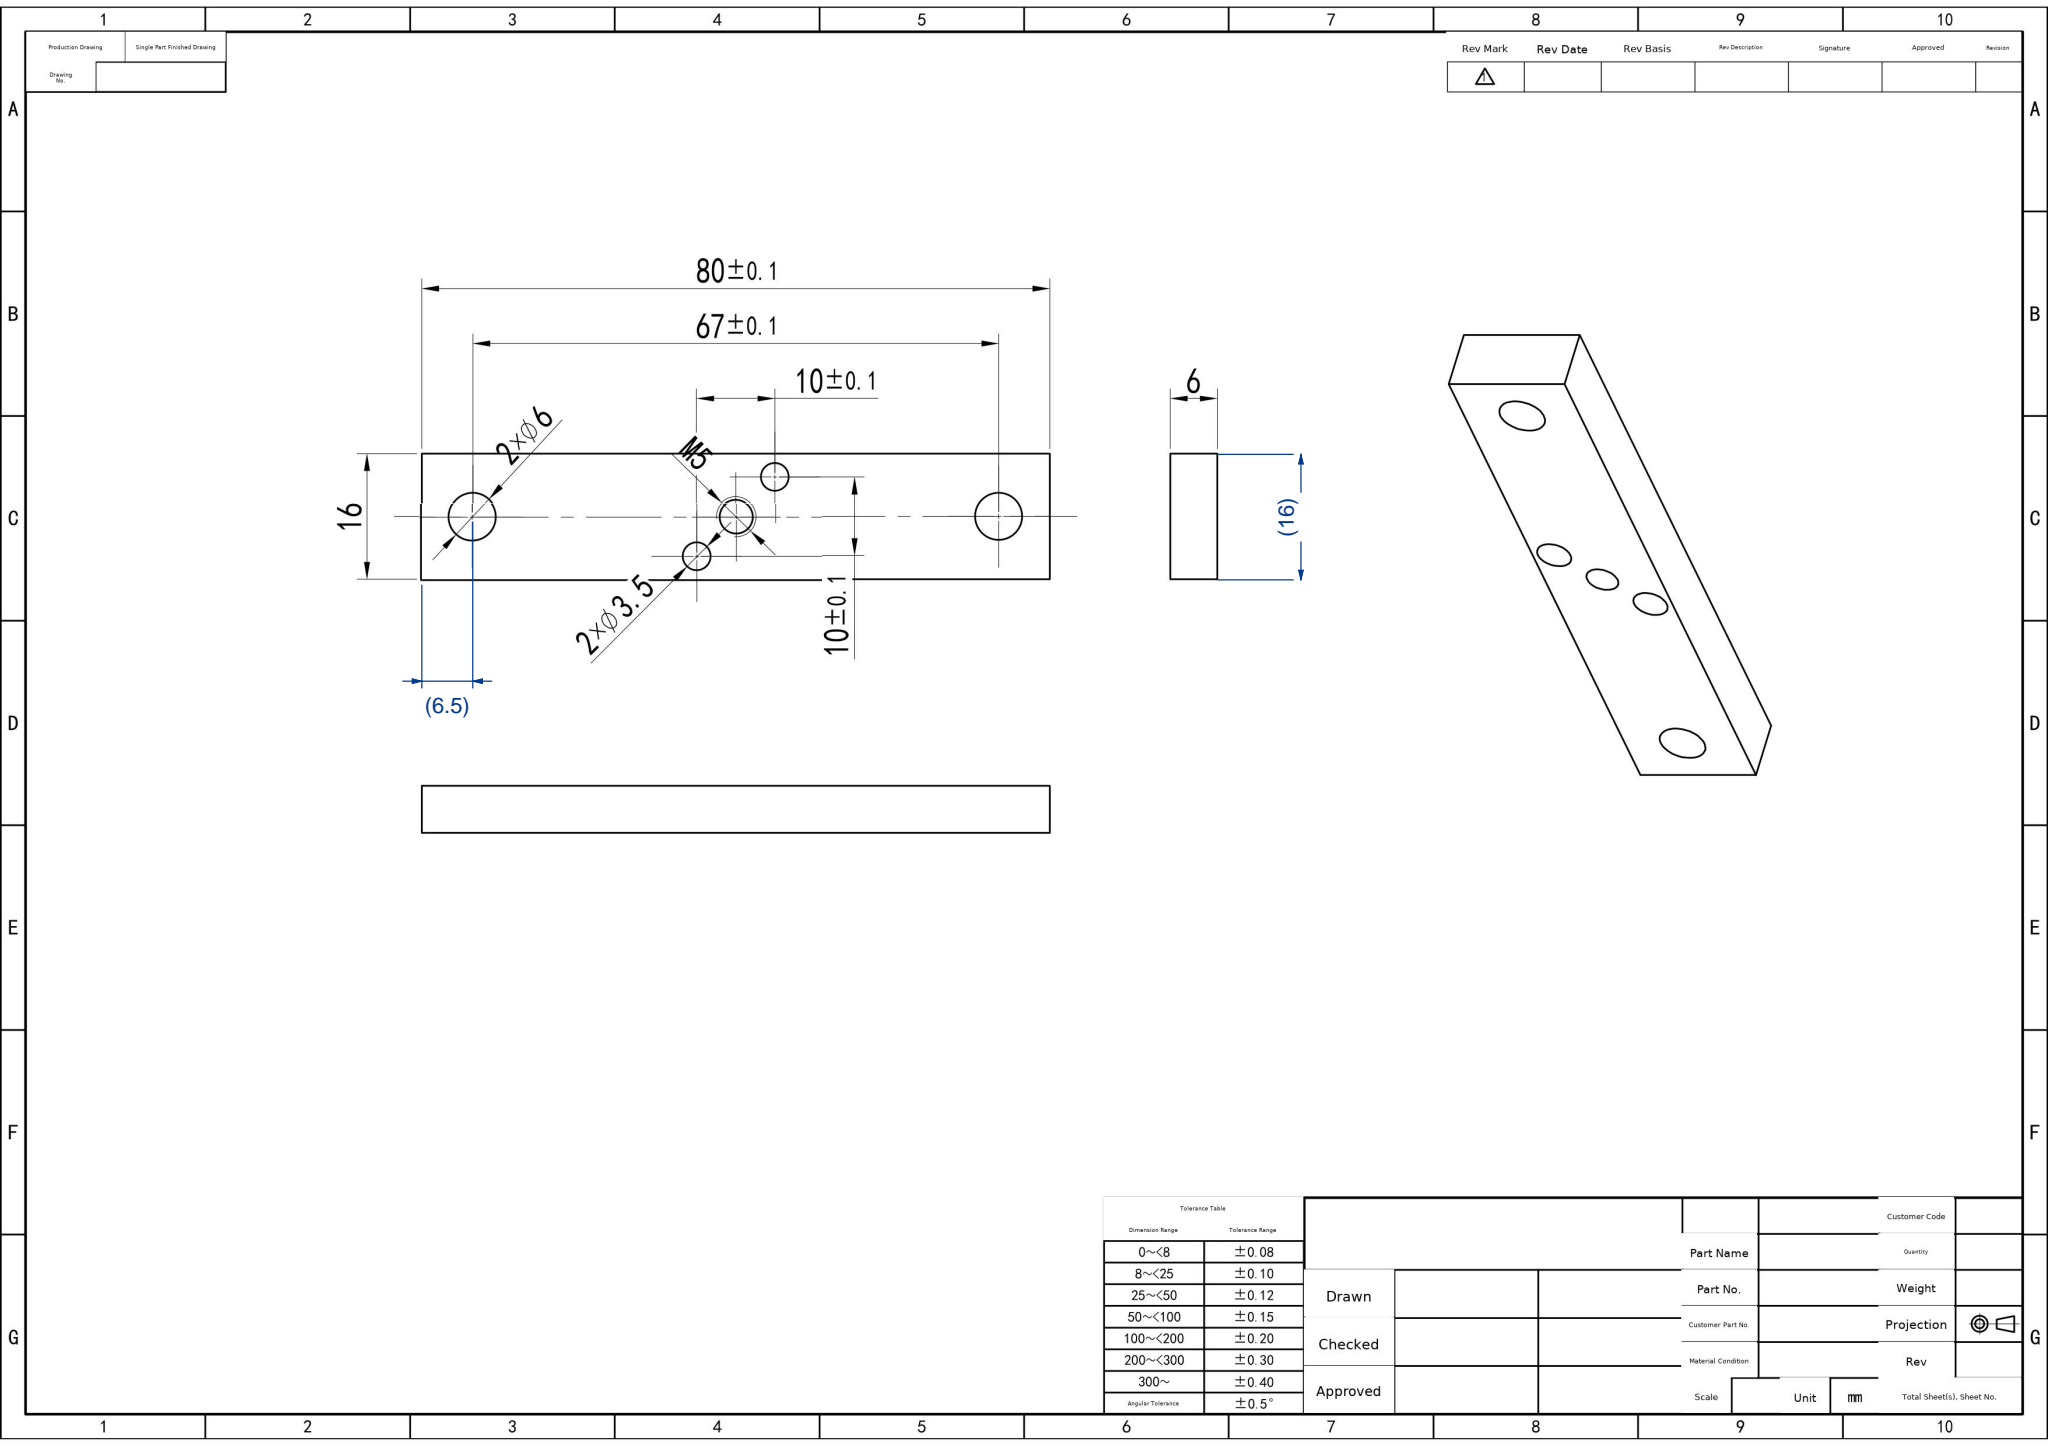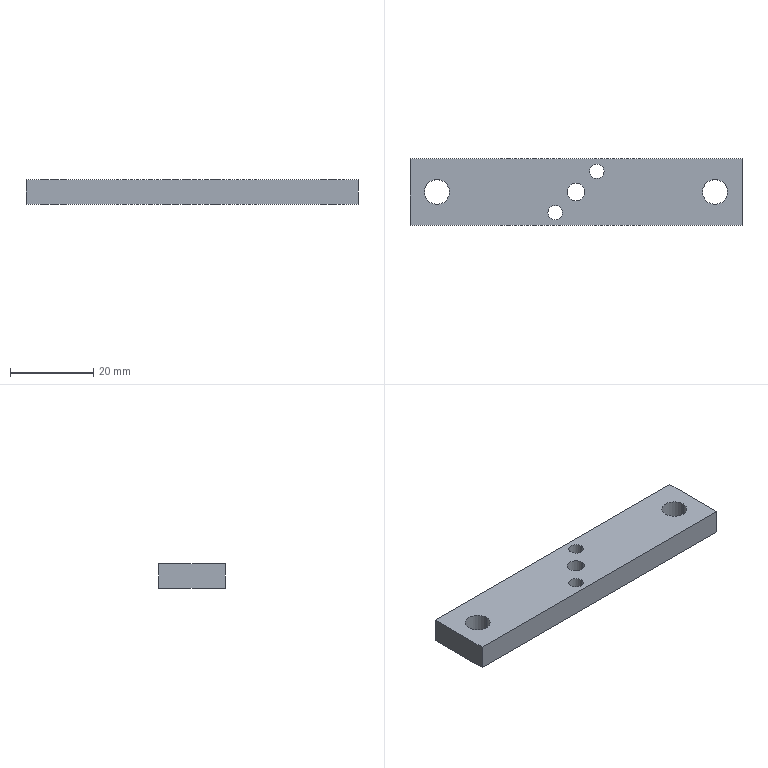Part | SolidWorks | mm | 1 solid | 16 faces | box 80 x 16 x 6 mm | volume 7142 mm3 | cylinder 10 | plane 6 | commonest cylinder face diameters 6 x4 3.5 x4 4.2 x2
STEP:
#1=CARTESIAN_POINT('',(36.5,0.,3.));
#2=VERTEX_POINT('',#1);
#3=CARTESIAN_POINT('',(30.5,0.,3.));
#4=VERTEX_POINT('',#3);
#5=CARTESIAN_POINT('',(33.5,0.,3.));
#6=DIRECTION('',(0.,0.,-1.));
#7=DIRECTION('',(-1.,0.,0.));
#8=AXIS2_PLACEMENT_3D('',#5,#6,#7);
#9=CIRCLE('',#8,3.);
#10=EDGE_CURVE('',#2,#4,#9,.T.);
#11=ORIENTED_EDGE('',*,*,#10,.F.);
#12=CARTESIAN_POINT('',(36.5,0.,-3.));
#13=VERTEX_POINT('',#12);
#14=CARTESIAN_POINT('',(36.5,0.,3.));
#15=DIRECTION('',(0.,0.,-1.));
#16=VECTOR('',#15,1000.);
#17=LINE('',#14,#16);
#18=EDGE_CURVE('',#2,#13,#17,.T.);
#19=ORIENTED_EDGE('',*,*,#18,.T.);
#20=CARTESIAN_POINT('',(30.5,0.,-3.));
#21=VERTEX_POINT('',#20);
#22=CARTESIAN_POINT('',(33.5,0.,-3.));
#23=DIRECTION('',(0.,0.,1.));
#24=DIRECTION('',(-1.,0.,0.));
#25=AXIS2_PLACEMENT_3D('',#22,#23,#24);
#26=CIRCLE('',#25,3.);
#27=EDGE_CURVE('',#21,#13,#26,.T.);
#28=ORIENTED_EDGE('',*,*,#27,.F.);
#29=CARTESIAN_POINT('',(30.5,0.,3.));
#30=DIRECTION('',(0.,0.,-1.));
#31=VECTOR('',#30,1000.);
#32=LINE('',#29,#31);
#33=EDGE_CURVE('',#4,#21,#32,.T.);
#34=ORIENTED_EDGE('',*,*,#33,.F.);
#35=EDGE_LOOP('',(#11,#19,#28,#34));
#36=FACE_OUTER_BOUND('',#35,.T.);
#37=CARTESIAN_POINT('',(33.5,0.,3.));
#38=DIRECTION('',(0.,0.,-1.));
#39=DIRECTION('',(-1.,0.,0.));
#40=AXIS2_PLACEMENT_3D('',#37,#38,#39);
#41=CYLINDRICAL_SURFACE('',#40,3.);
#42=ADVANCED_FACE('',(#36),#41,.F.);
#43=CARTESIAN_POINT('',(6.75,5.,3.));
#44=VERTEX_POINT('',#43);
#45=CARTESIAN_POINT('',(3.25,5.,3.));
#46=VERTEX_POINT('',#45);
#47=CARTESIAN_POINT('',(5.,5.,3.));
#48=DIRECTION('',(0.,0.,-1.));
#49=DIRECTION('',(-1.,0.,0.));
#50=AXIS2_PLACEMENT_3D('',#47,#48,#49);
#51=CIRCLE('',#50,1.75);
#52=EDGE_CURVE('',#44,#46,#51,.T.);
#53=ORIENTED_EDGE('',*,*,#52,.F.);
#54=CARTESIAN_POINT('',(6.75,5.,-3.));
#55=VERTEX_POINT('',#54);
#56=CARTESIAN_POINT('',(6.75,5.,3.));
#57=DIRECTION('',(0.,0.,-1.));
#58=VECTOR('',#57,1000.);
#59=LINE('',#56,#58);
#60=EDGE_CURVE('',#44,#55,#59,.T.);
#61=ORIENTED_EDGE('',*,*,#60,.T.);
#62=CARTESIAN_POINT('',(3.25,5.,-3.));
#63=VERTEX_POINT('',#62);
#64=CARTESIAN_POINT('',(5.,5.,-3.));
#65=DIRECTION('',(0.,0.,1.));
#66=DIRECTION('',(-1.,0.,0.));
#67=AXIS2_PLACEMENT_3D('',#64,#65,#66);
#68=CIRCLE('',#67,1.75);
#69=EDGE_CURVE('',#63,#55,#68,.T.);
#70=ORIENTED_EDGE('',*,*,#69,.F.);
#71=CARTESIAN_POINT('',(3.25,5.,3.));
#72=DIRECTION('',(0.,0.,-1.));
#73=VECTOR('',#72,1000.);
#74=LINE('',#71,#73);
#75=EDGE_CURVE('',#46,#63,#74,.T.);
#76=ORIENTED_EDGE('',*,*,#75,.F.);
#77=EDGE_LOOP('',(#53,#61,#70,#76));
#78=FACE_OUTER_BOUND('',#77,.T.);
#79=CARTESIAN_POINT('',(5.,5.,3.));
#80=DIRECTION('',(0.,0.,-1.));
#81=DIRECTION('',(-1.,0.,0.));
#82=AXIS2_PLACEMENT_3D('',#79,#80,#81);
#83=CYLINDRICAL_SURFACE('',#82,1.75);
#84=ADVANCED_FACE('',(#78),#83,.F.);
#85=CARTESIAN_POINT('',(2.1,0.,3.));
#86=VERTEX_POINT('',#85);
#87=CARTESIAN_POINT('',(-2.1,0.,3.));
#88=VERTEX_POINT('',#87);
#89=CARTESIAN_POINT('',(0.,0.,3.));
#90=DIRECTION('',(0.,0.,-1.));
#91=DIRECTION('',(-1.,0.,0.));
#92=AXIS2_PLACEMENT_3D('',#89,#90,#91);
#93=CIRCLE('',#92,2.1);
#94=EDGE_CURVE('',#86,#88,#93,.T.);
#95=ORIENTED_EDGE('',*,*,#94,.F.);
#96=CARTESIAN_POINT('',(2.1,0.,-3.));
#97=VERTEX_POINT('',#96);
#98=CARTESIAN_POINT('',(2.1,0.,3.));
#99=DIRECTION('',(0.,0.,-1.));
#100=VECTOR('',#99,1000.);
#101=LINE('',#98,#100);
#102=EDGE_CURVE('',#86,#97,#101,.T.);
#103=ORIENTED_EDGE('',*,*,#102,.T.);
#104=CARTESIAN_POINT('',(-2.1,0.,-3.));
#105=VERTEX_POINT('',#104);
#106=CARTESIAN_POINT('',(0.,0.,-3.));
#107=DIRECTION('',(0.,0.,1.));
#108=DIRECTION('',(-1.,0.,0.));
#109=AXIS2_PLACEMENT_3D('',#106,#107,#108);
#110=CIRCLE('',#109,2.1);
#111=EDGE_CURVE('',#105,#97,#110,.T.);
#112=ORIENTED_EDGE('',*,*,#111,.F.);
#113=CARTESIAN_POINT('',(-2.1,0.,3.));
#114=DIRECTION('',(0.,0.,-1.));
#115=VECTOR('',#114,1000.);
#116=LINE('',#113,#115);
#117=EDGE_CURVE('',#88,#105,#116,.T.);
#118=ORIENTED_EDGE('',*,*,#117,.F.);
#119=EDGE_LOOP('',(#95,#103,#112,#118));
#120=FACE_OUTER_BOUND('',#119,.T.);
#121=CARTESIAN_POINT('',(0.,0.,3.));
#122=DIRECTION('',(0.,0.,-1.));
#123=DIRECTION('',(-1.,0.,0.));
#124=AXIS2_PLACEMENT_3D('',#121,#122,#123);
#125=CYLINDRICAL_SURFACE('',#124,2.1);
#126=ADVANCED_FACE('',(#120),#125,.F.);
#127=CARTESIAN_POINT('',(-3.25,-5.,3.));
#128=VERTEX_POINT('',#127);
#129=CARTESIAN_POINT('',(-6.75,-5.,3.));
#130=VERTEX_POINT('',#129);
#131=CARTESIAN_POINT('',(-5.,-5.,3.));
#132=DIRECTION('',(0.,0.,-1.));
#133=DIRECTION('',(-1.,0.,0.));
#134=AXIS2_PLACEMENT_3D('',#131,#132,#133);
#135=CIRCLE('',#134,1.75);
#136=EDGE_CURVE('',#128,#130,#135,.T.);
#137=ORIENTED_EDGE('',*,*,#136,.F.);
#138=CARTESIAN_POINT('',(-3.25,-5.,-3.));
#139=VERTEX_POINT('',#138);
#140=CARTESIAN_POINT('',(-3.25,-5.,3.));
#141=DIRECTION('',(0.,0.,-1.));
#142=VECTOR('',#141,1000.);
#143=LINE('',#140,#142);
#144=EDGE_CURVE('',#128,#139,#143,.T.);
#145=ORIENTED_EDGE('',*,*,#144,.T.);
#146=CARTESIAN_POINT('',(-6.75,-5.,-3.));
#147=VERTEX_POINT('',#146);
#148=CARTESIAN_POINT('',(-5.,-5.,-3.));
#149=DIRECTION('',(0.,0.,1.));
#150=DIRECTION('',(-1.,0.,0.));
#151=AXIS2_PLACEMENT_3D('',#148,#149,#150);
#152=CIRCLE('',#151,1.75);
#153=EDGE_CURVE('',#147,#139,#152,.T.);
#154=ORIENTED_EDGE('',*,*,#153,.F.);
#155=CARTESIAN_POINT('',(-6.75,-5.,3.));
#156=DIRECTION('',(0.,0.,-1.));
#157=VECTOR('',#156,1000.);
#158=LINE('',#155,#157);
#159=EDGE_CURVE('',#130,#147,#158,.T.);
#160=ORIENTED_EDGE('',*,*,#159,.F.);
#161=EDGE_LOOP('',(#137,#145,#154,#160));
#162=FACE_OUTER_BOUND('',#161,.T.);
#163=CARTESIAN_POINT('',(-5.,-5.,3.));
#164=DIRECTION('',(0.,0.,-1.));
#165=DIRECTION('',(-1.,0.,0.));
#166=AXIS2_PLACEMENT_3D('',#163,#164,#165);
#167=CYLINDRICAL_SURFACE('',#166,1.75);
#168=ADVANCED_FACE('',(#162),#167,.F.);
#169=CARTESIAN_POINT('',(-30.5,0.,3.));
#170=VERTEX_POINT('',#169);
#171=CARTESIAN_POINT('',(-36.5,0.,3.));
#172=VERTEX_POINT('',#171);
#173=CARTESIAN_POINT('',(-33.5,0.,3.));
#174=DIRECTION('',(0.,0.,-1.));
#175=DIRECTION('',(-1.,0.,0.));
#176=AXIS2_PLACEMENT_3D('',#173,#174,#175);
#177=CIRCLE('',#176,3.);
#178=EDGE_CURVE('',#170,#172,#177,.T.);
#179=ORIENTED_EDGE('',*,*,#178,.F.);
#180=CARTESIAN_POINT('',(-30.5,0.,-3.));
#181=VERTEX_POINT('',#180);
#182=CARTESIAN_POINT('',(-30.5,0.,3.));
#183=DIRECTION('',(0.,0.,-1.));
#184=VECTOR('',#183,1000.);
#185=LINE('',#182,#184);
#186=EDGE_CURVE('',#170,#181,#185,.T.);
#187=ORIENTED_EDGE('',*,*,#186,.T.);
#188=CARTESIAN_POINT('',(-36.5,0.,-3.));
#189=VERTEX_POINT('',#188);
#190=CARTESIAN_POINT('',(-33.5,0.,-3.));
#191=DIRECTION('',(0.,0.,1.));
#192=DIRECTION('',(-1.,0.,0.));
#193=AXIS2_PLACEMENT_3D('',#190,#191,#192);
#194=CIRCLE('',#193,3.);
#195=EDGE_CURVE('',#189,#181,#194,.T.);
#196=ORIENTED_EDGE('',*,*,#195,.F.);
#197=CARTESIAN_POINT('',(-36.5,0.,3.));
#198=DIRECTION('',(0.,0.,-1.));
#199=VECTOR('',#198,1000.);
#200=LINE('',#197,#199);
#201=EDGE_CURVE('',#172,#189,#200,.T.);
#202=ORIENTED_EDGE('',*,*,#201,.F.);
#203=EDGE_LOOP('',(#179,#187,#196,#202));
#204=FACE_OUTER_BOUND('',#203,.T.);
#205=CARTESIAN_POINT('',(-33.5,0.,3.));
#206=DIRECTION('',(0.,0.,-1.));
#207=DIRECTION('',(-1.,0.,0.));
#208=AXIS2_PLACEMENT_3D('',#205,#206,#207);
#209=CYLINDRICAL_SURFACE('',#208,3.);
#210=ADVANCED_FACE('',(#204),#209,.F.);
#211=CARTESIAN_POINT('',(33.5,0.,3.));
#212=DIRECTION('',(0.,0.,-1.));
#213=DIRECTION('',(-1.,0.,0.));
#214=AXIS2_PLACEMENT_3D('',#211,#212,#213);
#215=CIRCLE('',#214,3.);
#216=EDGE_CURVE('',#4,#2,#215,.T.);
#217=ORIENTED_EDGE('',*,*,#216,.T.);
#218=ORIENTED_EDGE('',*,*,#10,.T.);
#219=EDGE_LOOP('',(#217,#218));
#220=FACE_BOUND('',#219,.T.);
#221=CARTESIAN_POINT('',(5.,5.,3.));
#222=DIRECTION('',(0.,0.,-1.));
#223=DIRECTION('',(-1.,0.,0.));
#224=AXIS2_PLACEMENT_3D('',#221,#222,#223);
#225=CIRCLE('',#224,1.75);
#226=EDGE_CURVE('',#46,#44,#225,.T.);
#227=ORIENTED_EDGE('',*,*,#226,.T.);
#228=ORIENTED_EDGE('',*,*,#52,.T.);
#229=EDGE_LOOP('',(#227,#228));
#230=FACE_BOUND('',#229,.T.);
#231=CARTESIAN_POINT('',(0.,0.,3.));
#232=DIRECTION('',(0.,0.,-1.));
#233=DIRECTION('',(-1.,0.,0.));
#234=AXIS2_PLACEMENT_3D('',#231,#232,#233);
#235=CIRCLE('',#234,2.1);
#236=EDGE_CURVE('',#88,#86,#235,.T.);
#237=ORIENTED_EDGE('',*,*,#236,.T.);
#238=ORIENTED_EDGE('',*,*,#94,.T.);
#239=EDGE_LOOP('',(#237,#238));
#240=FACE_BOUND('',#239,.T.);
#241=CARTESIAN_POINT('',(-5.,-5.,3.));
#242=DIRECTION('',(0.,0.,-1.));
#243=DIRECTION('',(-1.,0.,0.));
#244=AXIS2_PLACEMENT_3D('',#241,#242,#243);
#245=CIRCLE('',#244,1.75);
#246=EDGE_CURVE('',#130,#128,#245,.T.);
#247=ORIENTED_EDGE('',*,*,#246,.T.);
#248=ORIENTED_EDGE('',*,*,#136,.T.);
#249=EDGE_LOOP('',(#247,#248));
#250=FACE_BOUND('',#249,.T.);
#251=CARTESIAN_POINT('',(-33.5,0.,3.));
#252=DIRECTION('',(0.,0.,-1.));
#253=DIRECTION('',(-1.,0.,0.));
#254=AXIS2_PLACEMENT_3D('',#251,#252,#253);
#255=CIRCLE('',#254,3.);
#256=EDGE_CURVE('',#172,#170,#255,.T.);
#257=ORIENTED_EDGE('',*,*,#256,.T.);
#258=ORIENTED_EDGE('',*,*,#178,.T.);
#259=EDGE_LOOP('',(#257,#258));
#260=FACE_BOUND('',#259,.T.);
#261=CARTESIAN_POINT('',(40.,-8.,3.));
#262=VERTEX_POINT('',#261);
#263=CARTESIAN_POINT('',(40.,8.,3.));
#264=VERTEX_POINT('',#263);
#265=CARTESIAN_POINT('',(40.,0.,3.));
#266=DIRECTION('',(0.,1.,0.));
#267=VECTOR('',#266,1000.);
#268=LINE('',#265,#267);
#269=EDGE_CURVE('',#262,#264,#268,.T.);
#270=ORIENTED_EDGE('',*,*,#269,.T.);
#271=CARTESIAN_POINT('',(-40.,8.,3.));
#272=VERTEX_POINT('',#271);
#273=CARTESIAN_POINT('',(-33.5,8.,3.));
#274=DIRECTION('',(-1.,0.,0.));
#275=VECTOR('',#274,1000.);
#276=LINE('',#273,#275);
#277=EDGE_CURVE('',#264,#272,#276,.T.);
#278=ORIENTED_EDGE('',*,*,#277,.T.);
#279=CARTESIAN_POINT('',(-40.,-8.,3.));
#280=VERTEX_POINT('',#279);
#281=CARTESIAN_POINT('',(-40.,0.,3.));
#282=DIRECTION('',(0.,-1.,0.));
#283=VECTOR('',#282,1000.);
#284=LINE('',#281,#283);
#285=EDGE_CURVE('',#272,#280,#284,.T.);
#286=ORIENTED_EDGE('',*,*,#285,.T.);
#287=CARTESIAN_POINT('',(-33.5,-8.,3.));
#288=DIRECTION('',(1.,0.,0.));
#289=VECTOR('',#288,1000.);
#290=LINE('',#287,#289);
#291=EDGE_CURVE('',#280,#262,#290,.T.);
#292=ORIENTED_EDGE('',*,*,#291,.T.);
#293=EDGE_LOOP('',(#270,#278,#286,#292));
#294=FACE_OUTER_BOUND('',#293,.T.);
#295=CARTESIAN_POINT('',(-33.5,0.,3.));
#296=DIRECTION('',(0.,0.,1.));
#297=DIRECTION('',(1.,0.,0.));
#298=AXIS2_PLACEMENT_3D('',#295,#296,#297);
#299=PLANE('',#298);
#300=ADVANCED_FACE('',(#220,#230,#240,#250,#260,#294),#299,.T.);
#301=ORIENTED_EDGE('',*,*,#18,.F.);
#302=ORIENTED_EDGE('',*,*,#216,.F.);
#303=ORIENTED_EDGE('',*,*,#33,.T.);
#304=CARTESIAN_POINT('',(33.5,0.,-3.));
#305=DIRECTION('',(0.,0.,1.));
#306=DIRECTION('',(-1.,0.,0.));
#307=AXIS2_PLACEMENT_3D('',#304,#305,#306);
#308=CIRCLE('',#307,3.);
#309=EDGE_CURVE('',#13,#21,#308,.T.);
#310=ORIENTED_EDGE('',*,*,#309,.F.);
#311=EDGE_LOOP('',(#301,#302,#303,#310));
#312=FACE_OUTER_BOUND('',#311,.T.);
#313=CARTESIAN_POINT('',(33.5,0.,3.));
#314=DIRECTION('',(0.,0.,-1.));
#315=DIRECTION('',(-1.,0.,0.));
#316=AXIS2_PLACEMENT_3D('',#313,#314,#315);
#317=CYLINDRICAL_SURFACE('',#316,3.);
#318=ADVANCED_FACE('',(#312),#317,.F.);
#319=ORIENTED_EDGE('',*,*,#60,.F.);
#320=ORIENTED_EDGE('',*,*,#226,.F.);
#321=ORIENTED_EDGE('',*,*,#75,.T.);
#322=CARTESIAN_POINT('',(5.,5.,-3.));
#323=DIRECTION('',(0.,0.,1.));
#324=DIRECTION('',(-1.,0.,0.));
#325=AXIS2_PLACEMENT_3D('',#322,#323,#324);
#326=CIRCLE('',#325,1.75);
#327=EDGE_CURVE('',#55,#63,#326,.T.);
#328=ORIENTED_EDGE('',*,*,#327,.F.);
#329=EDGE_LOOP('',(#319,#320,#321,#328));
#330=FACE_OUTER_BOUND('',#329,.T.);
#331=CARTESIAN_POINT('',(5.,5.,3.));
#332=DIRECTION('',(0.,0.,-1.));
#333=DIRECTION('',(-1.,0.,0.));
#334=AXIS2_PLACEMENT_3D('',#331,#332,#333);
#335=CYLINDRICAL_SURFACE('',#334,1.75);
#336=ADVANCED_FACE('',(#330),#335,.F.);
#337=ORIENTED_EDGE('',*,*,#102,.F.);
#338=ORIENTED_EDGE('',*,*,#236,.F.);
#339=ORIENTED_EDGE('',*,*,#117,.T.);
#340=CARTESIAN_POINT('',(0.,0.,-3.));
#341=DIRECTION('',(0.,0.,1.));
#342=DIRECTION('',(-1.,0.,0.));
#343=AXIS2_PLACEMENT_3D('',#340,#341,#342);
#344=CIRCLE('',#343,2.1);
#345=EDGE_CURVE('',#97,#105,#344,.T.);
#346=ORIENTED_EDGE('',*,*,#345,.F.);
#347=EDGE_LOOP('',(#337,#338,#339,#346));
#348=FACE_OUTER_BOUND('',#347,.T.);
#349=CARTESIAN_POINT('',(0.,0.,3.));
#350=DIRECTION('',(0.,0.,-1.));
#351=DIRECTION('',(-1.,0.,0.));
#352=AXIS2_PLACEMENT_3D('',#349,#350,#351);
#353=CYLINDRICAL_SURFACE('',#352,2.1);
#354=ADVANCED_FACE('',(#348),#353,.F.);
#355=ORIENTED_EDGE('',*,*,#144,.F.);
#356=ORIENTED_EDGE('',*,*,#246,.F.);
#357=ORIENTED_EDGE('',*,*,#159,.T.);
#358=CARTESIAN_POINT('',(-5.,-5.,-3.));
#359=DIRECTION('',(0.,0.,1.));
#360=DIRECTION('',(-1.,0.,0.));
#361=AXIS2_PLACEMENT_3D('',#358,#359,#360);
#362=CIRCLE('',#361,1.75);
#363=EDGE_CURVE('',#139,#147,#362,.T.);
#364=ORIENTED_EDGE('',*,*,#363,.F.);
#365=EDGE_LOOP('',(#355,#356,#357,#364));
#366=FACE_OUTER_BOUND('',#365,.T.);
#367=CARTESIAN_POINT('',(-5.,-5.,3.));
#368=DIRECTION('',(0.,0.,-1.));
#369=DIRECTION('',(-1.,0.,0.));
#370=AXIS2_PLACEMENT_3D('',#367,#368,#369);
#371=CYLINDRICAL_SURFACE('',#370,1.75);
#372=ADVANCED_FACE('',(#366),#371,.F.);
#373=ORIENTED_EDGE('',*,*,#186,.F.);
#374=ORIENTED_EDGE('',*,*,#256,.F.);
#375=ORIENTED_EDGE('',*,*,#201,.T.);
#376=CARTESIAN_POINT('',(-33.5,0.,-3.));
#377=DIRECTION('',(0.,0.,1.));
#378=DIRECTION('',(-1.,0.,0.));
#379=AXIS2_PLACEMENT_3D('',#376,#377,#378);
#380=CIRCLE('',#379,3.);
#381=EDGE_CURVE('',#181,#189,#380,.T.);
#382=ORIENTED_EDGE('',*,*,#381,.F.);
#383=EDGE_LOOP('',(#373,#374,#375,#382));
#384=FACE_OUTER_BOUND('',#383,.T.);
#385=CARTESIAN_POINT('',(-33.5,0.,3.));
#386=DIRECTION('',(0.,0.,-1.));
#387=DIRECTION('',(-1.,0.,0.));
#388=AXIS2_PLACEMENT_3D('',#385,#386,#387);
#389=CYLINDRICAL_SURFACE('',#388,3.);
#390=ADVANCED_FACE('',(#384),#389,.F.);
#391=CARTESIAN_POINT('',(-40.,8.,-3.));
#392=VERTEX_POINT('',#391);
#393=CARTESIAN_POINT('',(-40.,8.,3.));
#394=DIRECTION('',(0.,0.,-1.));
#395=VECTOR('',#394,1000.);
#396=LINE('',#393,#395);
#397=EDGE_CURVE('',#272,#392,#396,.T.);
#398=ORIENTED_EDGE('',*,*,#397,.F.);
#399=ORIENTED_EDGE('',*,*,#277,.F.);
#400=CARTESIAN_POINT('',(40.,8.,-3.));
#401=VERTEX_POINT('',#400);
#402=CARTESIAN_POINT('',(40.,8.,3.));
#403=DIRECTION('',(0.,0.,1.));
#404=VECTOR('',#403,1000.);
#405=LINE('',#402,#404);
#406=EDGE_CURVE('',#401,#264,#405,.T.);
#407=ORIENTED_EDGE('',*,*,#406,.F.);
#408=CARTESIAN_POINT('',(40.,8.,-3.));
#409=DIRECTION('',(1.,0.,0.));
#410=VECTOR('',#409,1000.);
#411=LINE('',#408,#410);
#412=EDGE_CURVE('',#392,#401,#411,.T.);
#413=ORIENTED_EDGE('',*,*,#412,.F.);
#414=EDGE_LOOP('',(#398,#399,#407,#413));
#415=FACE_OUTER_BOUND('',#414,.T.);
#416=CARTESIAN_POINT('',(40.,8.,3.));
#417=DIRECTION('',(0.,-1.,0.));
#418=DIRECTION('',(0.,0.,-1.));
#419=AXIS2_PLACEMENT_3D('',#416,#417,#418);
#420=PLANE('',#419);
#421=ADVANCED_FACE('',(#415),#420,.F.);
#422=ORIENTED_EDGE('',*,*,#406,.T.);
#423=ORIENTED_EDGE('',*,*,#269,.F.);
#424=CARTESIAN_POINT('',(40.,-8.,-3.));
#425=VERTEX_POINT('',#424);
#426=CARTESIAN_POINT('',(40.,-8.,3.));
#427=DIRECTION('',(0.,0.,1.));
#428=VECTOR('',#427,1000.);
#429=LINE('',#426,#428);
#430=EDGE_CURVE('',#425,#262,#429,.T.);
#431=ORIENTED_EDGE('',*,*,#430,.F.);
#432=CARTESIAN_POINT('',(40.,-8.,-3.));
#433=DIRECTION('',(0.,-1.,0.));
#434=VECTOR('',#433,1000.);
#435=LINE('',#432,#434);
#436=EDGE_CURVE('',#401,#425,#435,.T.);
#437=ORIENTED_EDGE('',*,*,#436,.F.);
#438=EDGE_LOOP('',(#422,#423,#431,#437));
#439=FACE_OUTER_BOUND('',#438,.T.);
#440=CARTESIAN_POINT('',(40.,-8.,3.));
#441=DIRECTION('',(-1.,0.,0.));
#442=DIRECTION('',(0.,0.,1.));
#443=AXIS2_PLACEMENT_3D('',#440,#441,#442);
#444=PLANE('',#443);
#445=ADVANCED_FACE('',(#439),#444,.F.);
#446=ORIENTED_EDGE('',*,*,#430,.T.);
#447=ORIENTED_EDGE('',*,*,#291,.F.);
#448=CARTESIAN_POINT('',(-40.,-8.,-3.));
#449=VERTEX_POINT('',#448);
#450=CARTESIAN_POINT('',(-40.,-8.,3.));
#451=DIRECTION('',(0.,0.,1.));
#452=VECTOR('',#451,1000.);
#453=LINE('',#450,#452);
#454=EDGE_CURVE('',#449,#280,#453,.T.);
#455=ORIENTED_EDGE('',*,*,#454,.F.);
#456=CARTESIAN_POINT('',(-40.,-8.,-3.));
#457=DIRECTION('',(-1.,0.,0.));
#458=VECTOR('',#457,1000.);
#459=LINE('',#456,#458);
#460=EDGE_CURVE('',#425,#449,#459,.T.);
#461=ORIENTED_EDGE('',*,*,#460,.F.);
#462=EDGE_LOOP('',(#446,#447,#455,#461));
#463=FACE_OUTER_BOUND('',#462,.T.);
#464=CARTESIAN_POINT('',(-40.,-8.,3.));
#465=DIRECTION('',(0.,1.,0.));
#466=DIRECTION('',(0.,0.,1.));
#467=AXIS2_PLACEMENT_3D('',#464,#465,#466);
#468=PLANE('',#467);
#469=ADVANCED_FACE('',(#463),#468,.F.);
#470=ORIENTED_EDGE('',*,*,#454,.T.);
#471=ORIENTED_EDGE('',*,*,#285,.F.);
#472=ORIENTED_EDGE('',*,*,#397,.T.);
#473=CARTESIAN_POINT('',(-40.,8.,-3.));
#474=DIRECTION('',(0.,1.,0.));
#475=VECTOR('',#474,1000.);
#476=LINE('',#473,#475);
#477=EDGE_CURVE('',#449,#392,#476,.T.);
#478=ORIENTED_EDGE('',*,*,#477,.F.);
#479=EDGE_LOOP('',(#470,#471,#472,#478));
#480=FACE_OUTER_BOUND('',#479,.T.);
#481=CARTESIAN_POINT('',(-40.,8.,3.));
#482=DIRECTION('',(1.,0.,0.));
#483=DIRECTION('',(0.,0.,-1.));
#484=AXIS2_PLACEMENT_3D('',#481,#482,#483);
#485=PLANE('',#484);
#486=ADVANCED_FACE('',(#480),#485,.F.);
#487=ORIENTED_EDGE('',*,*,#27,.T.);
#488=ORIENTED_EDGE('',*,*,#309,.T.);
#489=EDGE_LOOP('',(#487,#488));
#490=FACE_BOUND('',#489,.T.);
#491=ORIENTED_EDGE('',*,*,#69,.T.);
#492=ORIENTED_EDGE('',*,*,#327,.T.);
#493=EDGE_LOOP('',(#491,#492));
#494=FACE_BOUND('',#493,.T.);
#495=ORIENTED_EDGE('',*,*,#111,.T.);
#496=ORIENTED_EDGE('',*,*,#345,.T.);
#497=EDGE_LOOP('',(#495,#496));
#498=FACE_BOUND('',#497,.T.);
#499=ORIENTED_EDGE('',*,*,#153,.T.);
#500=ORIENTED_EDGE('',*,*,#363,.T.);
#501=EDGE_LOOP('',(#499,#500));
#502=FACE_BOUND('',#501,.T.);
#503=ORIENTED_EDGE('',*,*,#195,.T.);
#504=ORIENTED_EDGE('',*,*,#381,.T.);
#505=EDGE_LOOP('',(#503,#504));
#506=FACE_BOUND('',#505,.T.);
#507=ORIENTED_EDGE('',*,*,#412,.T.);
#508=ORIENTED_EDGE('',*,*,#436,.T.);
#509=ORIENTED_EDGE('',*,*,#460,.T.);
#510=ORIENTED_EDGE('',*,*,#477,.T.);
#511=EDGE_LOOP('',(#507,#508,#509,#510));
#512=FACE_OUTER_BOUND('',#511,.T.);
#513=CARTESIAN_POINT('',(-33.5,0.,-3.));
#514=DIRECTION('',(0.,0.,1.));
#515=DIRECTION('',(1.,0.,0.));
#516=AXIS2_PLACEMENT_3D('',#513,#514,#515);
#517=PLANE('',#516);
#518=ADVANCED_FACE('',(#490,#494,#498,#502,#506,#512),#517,.F.);
#519=CLOSED_SHELL('',(#42,#84,#126,#168,#210,#300,#318,#336,#354,#372,#390,#421,#445,#469,#486,#518));
#520=MANIFOLD_SOLID_BREP('',#519);
#521=CARTESIAN_POINT('',(0.,0.,0.));
#522=DIRECTION('',(0.,0.,1.));
#523=DIRECTION('',(1.,0.,0.));
#524=AXIS2_PLACEMENT_3D('',#521,#522,#523);
#525=(LENGTH_UNIT()NAMED_UNIT(*)SI_UNIT(.MILLI.,.METRE.));
#526=UNCERTAINTY_MEASURE_WITH_UNIT(LENGTH_MEASURE(0.00001),#525,'','');
#527=(NAMED_UNIT(*)PLANE_ANGLE_UNIT()SI_UNIT($,.RADIAN.));
#528=(NAMED_UNIT(*)SI_UNIT($,.STERADIAN.)SOLID_ANGLE_UNIT());
#529=(GEOMETRIC_REPRESENTATION_CONTEXT(3)GLOBAL_UNCERTAINTY_ASSIGNED_CONTEXT((#526))GLOBAL_UNIT_ASSIGNED_CONTEXT((#525,#527,#528))REPRESENTATION_CONTEXT('',''));
#530=ADVANCED_BREP_SHAPE_REPRESENTATION('',(#520,#524),#529);